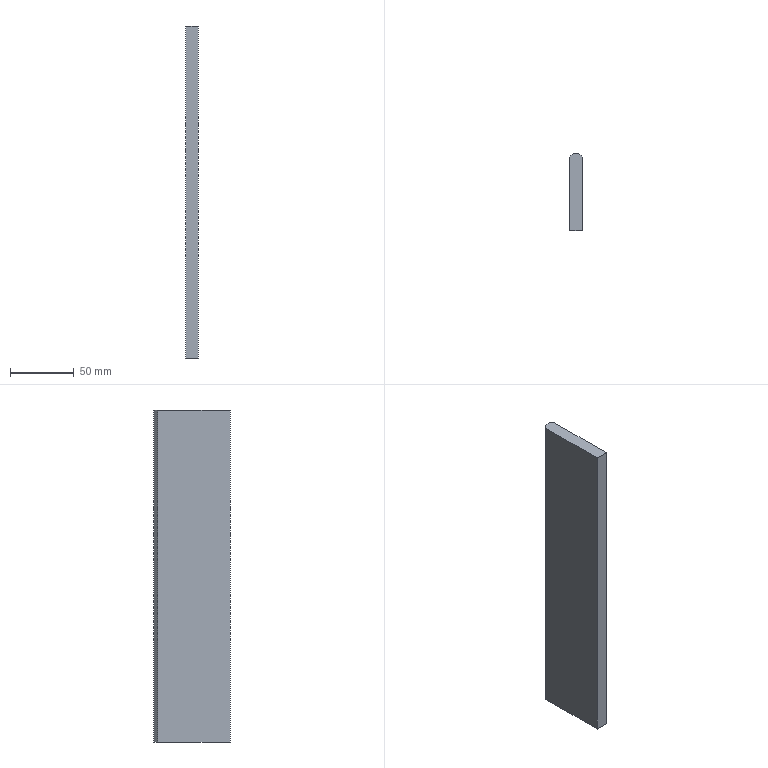Component | SolidWorks | JigBaffle-1 | 1 solid | 8 faces | box 10 x 60 x 260 mm | volume 153660 mm3 | plane 8 | material Copper
build123d program:
from build123d import *

# Parameters (mm, degrees)
SKETCH1_W           = 10
SKETCH1_H           = 60
BOSS_EXTRUDE1_DEPTH = 260
CHAMFER1_SIZE       = 3


with BuildPart() as part:
    # Sketch1 → Boss-Extrude1 (new body)
    with BuildSketch(Plane.XY):
        with Locations((5, 30)):
            Rectangle(SKETCH1_W, SKETCH1_H)
    extrude(amount=BOSS_EXTRUDE1_DEPTH)

    # Chamfer1
    chamfer1_edges = [part.edges().sort_by_distance(p)[0] for p in [
        (0, 60, 130),
        (10, 60, 130),
    ]]
    chamfer(chamfer1_edges, length=CHAMFER1_SIZE)


solid = part.part

# Placed as in the assembly
solid = solid.moved(Location((51.992, -107.909, 1070), (0, 0, 0)))
STEP:
#1=COLOUR_RGB('',0.7922,0.8196,0.9333);
#2=FILL_AREA_STYLE_COLOUR('',#1);
#3=FILL_AREA_STYLE('',(#2));
#4=SURFACE_STYLE_FILL_AREA(#3);
#5=SURFACE_SIDE_STYLE('',(#4));
#6=SURFACE_STYLE_USAGE(.BOTH.,#5);
#7=PRESENTATION_STYLE_ASSIGNMENT((#6));
#8=CARTESIAN_POINT('',(2.047,-2.004,52.362));
#9=VERTEX_POINT('',#8);
#10=CARTESIAN_POINT('',(2.047,-4.248,52.362));
#11=VERTEX_POINT('',#10);
#12=CARTESIAN_POINT('',(2.047,-4.248,52.362));
#13=DIRECTION('',(0.,-1.,0.));
#14=VECTOR('',#13,39.37);
#15=LINE('',#12,#14);
#16=EDGE_CURVE('',#9,#11,#15,.T.);
#17=ORIENTED_EDGE('',*,*,#16,.F.);
#18=CARTESIAN_POINT('',(2.047,-2.004,42.126));
#19=VERTEX_POINT('',#18);
#20=CARTESIAN_POINT('',(2.047,-2.004,52.362));
#21=DIRECTION('',(0.,0.,-1.));
#22=VECTOR('',#21,39.37);
#23=LINE('',#20,#22);
#24=EDGE_CURVE('',#9,#19,#23,.T.);
#25=ORIENTED_EDGE('',*,*,#24,.T.);
#26=CARTESIAN_POINT('',(2.047,-4.248,42.126));
#27=VERTEX_POINT('',#26);
#28=CARTESIAN_POINT('',(2.047,-4.248,42.126));
#29=DIRECTION('',(0.,-1.,0.));
#30=VECTOR('',#29,39.37);
#31=LINE('',#28,#30);
#32=EDGE_CURVE('',#19,#27,#31,.T.);
#33=ORIENTED_EDGE('',*,*,#32,.T.);
#34=CARTESIAN_POINT('',(2.047,-4.248,52.362));
#35=DIRECTION('',(0.,0.,-1.));
#36=VECTOR('',#35,39.37);
#37=LINE('',#34,#36);
#38=EDGE_CURVE('',#11,#27,#37,.T.);
#39=ORIENTED_EDGE('',*,*,#38,.F.);
#40=EDGE_LOOP('',(#17,#25,#33,#39));
#41=FACE_OUTER_BOUND('',#40,.T.);
#42=CARTESIAN_POINT('',(2.047,-4.248,52.362));
#43=DIRECTION('',(1.,0.,0.));
#44=DIRECTION('',(0.,0.,-1.));
#45=AXIS2_PLACEMENT_3D('',#42,#43,#44);
#46=PLANE('',#45);
#47=ADVANCED_FACE('',(#41),#46,.F.);
#48=CARTESIAN_POINT('',(2.441,-4.248,42.126));
#49=VERTEX_POINT('',#48);
#50=CARTESIAN_POINT('',(2.047,-4.248,42.126));
#51=DIRECTION('',(1.,0.,0.));
#52=VECTOR('',#51,39.37);
#53=LINE('',#50,#52);
#54=EDGE_CURVE('',#27,#49,#53,.T.);
#55=ORIENTED_EDGE('',*,*,#54,.T.);
#56=CARTESIAN_POINT('',(2.441,-4.248,52.362));
#57=VERTEX_POINT('',#56);
#58=CARTESIAN_POINT('',(2.441,-4.248,52.362));
#59=DIRECTION('',(0.,0.,-1.));
#60=VECTOR('',#59,39.37);
#61=LINE('',#58,#60);
#62=EDGE_CURVE('',#57,#49,#61,.T.);
#63=ORIENTED_EDGE('',*,*,#62,.F.);
#64=CARTESIAN_POINT('',(2.047,-4.248,52.362));
#65=DIRECTION('',(1.,0.,0.));
#66=VECTOR('',#65,39.37);
#67=LINE('',#64,#66);
#68=EDGE_CURVE('',#11,#57,#67,.T.);
#69=ORIENTED_EDGE('',*,*,#68,.F.);
#70=ORIENTED_EDGE('',*,*,#38,.T.);
#71=EDGE_LOOP('',(#55,#63,#69,#70));
#72=FACE_OUTER_BOUND('',#71,.T.);
#73=CARTESIAN_POINT('',(2.047,-4.248,52.362));
#74=DIRECTION('',(0.,1.,0.));
#75=DIRECTION('',(0.,0.,1.));
#76=AXIS2_PLACEMENT_3D('',#73,#74,#75);
#77=PLANE('',#76);
#78=ADVANCED_FACE('',(#72),#77,.F.);
#79=CARTESIAN_POINT('',(2.441,-2.004,42.126));
#80=VERTEX_POINT('',#79);
#81=CARTESIAN_POINT('',(2.441,-4.248,42.126));
#82=DIRECTION('',(0.,1.,0.));
#83=VECTOR('',#82,39.37);
#84=LINE('',#81,#83);
#85=EDGE_CURVE('',#49,#80,#84,.T.);
#86=ORIENTED_EDGE('',*,*,#85,.T.);
#87=CARTESIAN_POINT('',(2.441,-2.004,52.362));
#88=VERTEX_POINT('',#87);
#89=CARTESIAN_POINT('',(2.441,-2.004,52.362));
#90=DIRECTION('',(0.,0.,1.));
#91=VECTOR('',#90,39.37);
#92=LINE('',#89,#91);
#93=EDGE_CURVE('',#80,#88,#92,.T.);
#94=ORIENTED_EDGE('',*,*,#93,.T.);
#95=CARTESIAN_POINT('',(2.441,-4.248,52.362));
#96=DIRECTION('',(0.,1.,0.));
#97=VECTOR('',#96,39.37);
#98=LINE('',#95,#97);
#99=EDGE_CURVE('',#57,#88,#98,.T.);
#100=ORIENTED_EDGE('',*,*,#99,.F.);
#101=ORIENTED_EDGE('',*,*,#62,.T.);
#102=EDGE_LOOP('',(#86,#94,#100,#101));
#103=FACE_OUTER_BOUND('',#102,.T.);
#104=CARTESIAN_POINT('',(2.441,-4.248,52.362));
#105=DIRECTION('',(-1.,0.,0.));
#106=DIRECTION('',(0.,0.,1.));
#107=AXIS2_PLACEMENT_3D('',#104,#105,#106);
#108=PLANE('',#107);
#109=ADVANCED_FACE('',(#103),#108,.F.);
#110=CARTESIAN_POINT('',(2.323,-1.886,42.126));
#111=VERTEX_POINT('',#110);
#112=CARTESIAN_POINT('',(2.165,-1.886,42.126));
#113=VERTEX_POINT('',#112);
#114=CARTESIAN_POINT('',(2.047,-1.886,42.126));
#115=DIRECTION('',(-1.,0.,0.));
#116=VECTOR('',#115,39.37);
#117=LINE('',#114,#116);
#118=EDGE_CURVE('',#111,#113,#117,.T.);
#119=ORIENTED_EDGE('',*,*,#118,.T.);
#120=CARTESIAN_POINT('',(2.165,-1.886,52.362));
#121=VERTEX_POINT('',#120);
#122=CARTESIAN_POINT('',(2.165,-1.886,52.362));
#123=DIRECTION('',(0.,0.,1.));
#124=VECTOR('',#123,39.37);
#125=LINE('',#122,#124);
#126=EDGE_CURVE('',#113,#121,#125,.T.);
#127=ORIENTED_EDGE('',*,*,#126,.T.);
#128=CARTESIAN_POINT('',(2.323,-1.886,52.362));
#129=VERTEX_POINT('',#128);
#130=CARTESIAN_POINT('',(2.047,-1.886,52.362));
#131=DIRECTION('',(-1.,0.,0.));
#132=VECTOR('',#131,39.37);
#133=LINE('',#130,#132);
#134=EDGE_CURVE('',#129,#121,#133,.T.);
#135=ORIENTED_EDGE('',*,*,#134,.F.);
#136=CARTESIAN_POINT('',(2.323,-1.886,52.362));
#137=DIRECTION('',(0.,0.,-1.));
#138=VECTOR('',#137,39.37);
#139=LINE('',#136,#138);
#140=EDGE_CURVE('',#129,#111,#139,.T.);
#141=ORIENTED_EDGE('',*,*,#140,.T.);
#142=EDGE_LOOP('',(#119,#127,#135,#141));
#143=FACE_OUTER_BOUND('',#142,.T.);
#144=CARTESIAN_POINT('',(2.047,-1.886,52.362));
#145=DIRECTION('',(0.,-1.,0.));
#146=DIRECTION('',(0.,0.,-1.));
#147=AXIS2_PLACEMENT_3D('',#144,#145,#146);
#148=PLANE('',#147);
#149=ADVANCED_FACE('',(#143),#148,.F.);
#150=ORIENTED_EDGE('',*,*,#134,.T.);
#151=CARTESIAN_POINT('',(2.047,-2.004,52.362));
#152=DIRECTION('',(-0.7071,-0.7071,0.));
#153=VECTOR('',#152,39.37);
#154=LINE('',#151,#153);
#155=EDGE_CURVE('',#121,#9,#154,.T.);
#156=ORIENTED_EDGE('',*,*,#155,.T.);
#157=ORIENTED_EDGE('',*,*,#16,.T.);
#158=ORIENTED_EDGE('',*,*,#68,.T.);
#159=ORIENTED_EDGE('',*,*,#99,.T.);
#160=CARTESIAN_POINT('',(2.323,-1.886,52.362));
#161=DIRECTION('',(-0.7071,0.7071,0.));
#162=VECTOR('',#161,39.37);
#163=LINE('',#160,#162);
#164=EDGE_CURVE('',#88,#129,#163,.T.);
#165=ORIENTED_EDGE('',*,*,#164,.T.);
#166=EDGE_LOOP('',(#150,#156,#157,#158,#159,#165));
#167=FACE_OUTER_BOUND('',#166,.T.);
#168=CARTESIAN_POINT('',(2.047,-4.248,52.362));
#169=DIRECTION('',(0.,0.,-1.));
#170=DIRECTION('',(-1.,0.,0.));
#171=AXIS2_PLACEMENT_3D('',#168,#169,#170);
#172=PLANE('',#171);
#173=ADVANCED_FACE('',(#167),#172,.F.);
#174=ORIENTED_EDGE('',*,*,#32,.F.);
#175=CARTESIAN_POINT('',(0.9249,-3.126,42.126));
#176=DIRECTION('',(0.7071,0.7071,0.));
#177=VECTOR('',#176,39.37);
#178=LINE('',#175,#177);
#179=EDGE_CURVE('',#19,#113,#178,.T.);
#180=ORIENTED_EDGE('',*,*,#179,.T.);
#181=ORIENTED_EDGE('',*,*,#118,.F.);
#182=CARTESIAN_POINT('',(3.366,-2.93,42.126));
#183=DIRECTION('',(0.7071,-0.7071,0.));
#184=VECTOR('',#183,39.37);
#185=LINE('',#182,#184);
#186=EDGE_CURVE('',#111,#80,#185,.T.);
#187=ORIENTED_EDGE('',*,*,#186,.T.);
#188=ORIENTED_EDGE('',*,*,#85,.F.);
#189=ORIENTED_EDGE('',*,*,#54,.F.);
#190=EDGE_LOOP('',(#174,#180,#181,#187,#188,#189));
#191=FACE_OUTER_BOUND('',#190,.T.);
#192=CARTESIAN_POINT('',(2.047,-4.248,42.126));
#193=DIRECTION('',(0.,0.,-1.));
#194=DIRECTION('',(-1.,0.,0.));
#195=AXIS2_PLACEMENT_3D('',#192,#193,#194);
#196=PLANE('',#195);
#197=ADVANCED_FACE('',(#191),#196,.T.);
#198=ORIENTED_EDGE('',*,*,#155,.F.);
#199=ORIENTED_EDGE('',*,*,#126,.F.);
#200=ORIENTED_EDGE('',*,*,#179,.F.);
#201=ORIENTED_EDGE('',*,*,#24,.F.);
#202=EDGE_LOOP('',(#198,#199,#200,#201));
#203=FACE_OUTER_BOUND('',#202,.T.);
#204=CARTESIAN_POINT('',(2.047,-2.004,52.362));
#205=DIRECTION('',(0.7071,-0.7071,0.));
#206=DIRECTION('',(0.,0.,-1.));
#207=AXIS2_PLACEMENT_3D('',#204,#205,#206);
#208=PLANE('',#207);
#209=ADVANCED_FACE('',(#203),#208,.F.);
#210=ORIENTED_EDGE('',*,*,#164,.F.);
#211=ORIENTED_EDGE('',*,*,#93,.F.);
#212=ORIENTED_EDGE('',*,*,#186,.F.);
#213=ORIENTED_EDGE('',*,*,#140,.F.);
#214=EDGE_LOOP('',(#210,#211,#212,#213));
#215=FACE_OUTER_BOUND('',#214,.T.);
#216=CARTESIAN_POINT('',(2.323,-1.886,52.362));
#217=DIRECTION('',(-0.7071,-0.7071,0.));
#218=DIRECTION('',(0.,0.,-1.));
#219=AXIS2_PLACEMENT_3D('',#216,#217,#218);
#220=PLANE('',#219);
#221=ADVANCED_FACE('',(#215),#220,.F.);
#222=CLOSED_SHELL('',(#47,#78,#109,#149,#173,#197,#209,#221));
#223=MANIFOLD_SOLID_BREP('',#222);
#224=STYLED_ITEM('',(#7),#223);
#225=PRESENTATION_LAYER_ASSIGNMENT('','',(#224));
#226=(LENGTH_UNIT()NAMED_UNIT(*)SI_UNIT($,.METRE.));
#227=LENGTH_MEASURE_WITH_UNIT(LENGTH_MEASURE(0.0254),#226);
#228=DIMENSIONAL_EXPONENTS(1.,0.,0.,0.,0.,0.,0.);
#229=(CONVERSION_BASED_UNIT('',#227)LENGTH_UNIT()NAMED_UNIT(#228));
#230=UNCERTAINTY_MEASURE_WITH_UNIT(LENGTH_MEASURE(0.00001),#229,'','');
#231=(NAMED_UNIT(*)PLANE_ANGLE_UNIT()SI_UNIT($,.RADIAN.));
#232=(NAMED_UNIT(*)SI_UNIT($,.STERADIAN.)SOLID_ANGLE_UNIT());
#233=(GEOMETRIC_REPRESENTATION_CONTEXT(3)GLOBAL_UNCERTAINTY_ASSIGNED_CONTEXT((#230))GLOBAL_UNIT_ASSIGNED_CONTEXT((#229,#231,#232))REPRESENTATION_CONTEXT('',''));
#234=MECHANICAL_DESIGN_GEOMETRIC_PRESENTATION_REPRESENTATION('',(#224),#233);
#235=CARTESIAN_POINT('',(0.,0.,0.));
#236=DIRECTION('',(0.,0.,1.));
#237=DIRECTION('',(1.,0.,0.));
#238=AXIS2_PLACEMENT_3D('',#235,#236,#237);
#239=(LENGTH_UNIT()NAMED_UNIT(*)SI_UNIT($,.METRE.));
#240=LENGTH_MEASURE_WITH_UNIT(LENGTH_MEASURE(0.0254),#239);
#241=DIMENSIONAL_EXPONENTS(1.,0.,0.,0.,0.,0.,0.);
#242=(CONVERSION_BASED_UNIT('',#240)LENGTH_UNIT()NAMED_UNIT(#241));
#243=UNCERTAINTY_MEASURE_WITH_UNIT(LENGTH_MEASURE(0.00001),#242,'','');
#244=(NAMED_UNIT(*)PLANE_ANGLE_UNIT()SI_UNIT($,.RADIAN.));
#245=(NAMED_UNIT(*)SI_UNIT($,.STERADIAN.)SOLID_ANGLE_UNIT());
#246=(GEOMETRIC_REPRESENTATION_CONTEXT(3)GLOBAL_UNCERTAINTY_ASSIGNED_CONTEXT((#243))GLOBAL_UNIT_ASSIGNED_CONTEXT((#242,#244,#245))REPRESENTATION_CONTEXT('',''));
#247=ADVANCED_BREP_SHAPE_REPRESENTATION('',(#223,#238),#246);